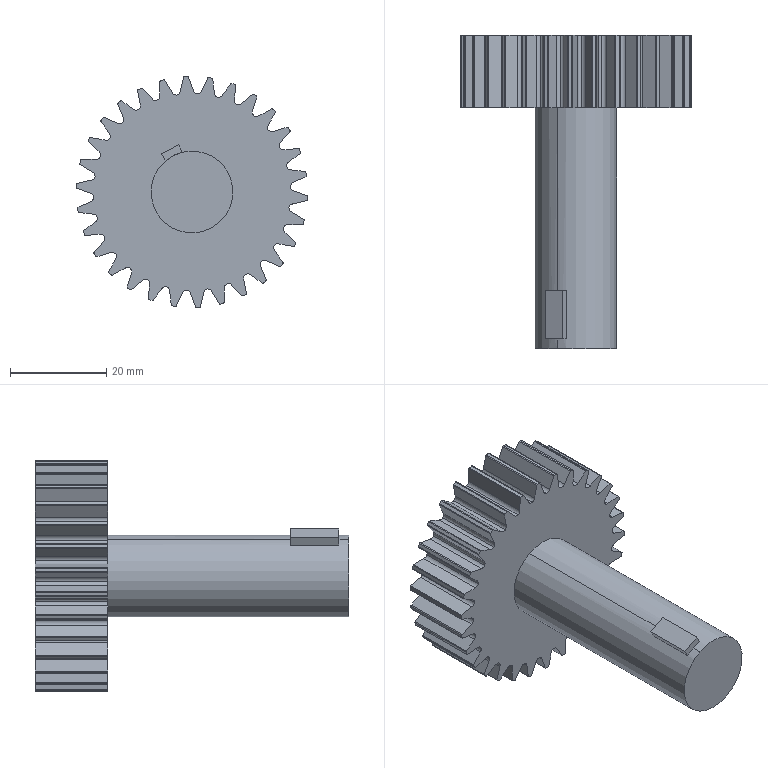Component | SolidWorks | Engrenange 30-1 | 1 solid | 235 faces | box 47.96 x 65 x 47.97 mm | volume 26303 mm3 | cylinder 166 | spline 60 | plane 9 | commonest cylinder face diameters 1.996 x71 0.4 x60 48 x31 34 x2 17 x2